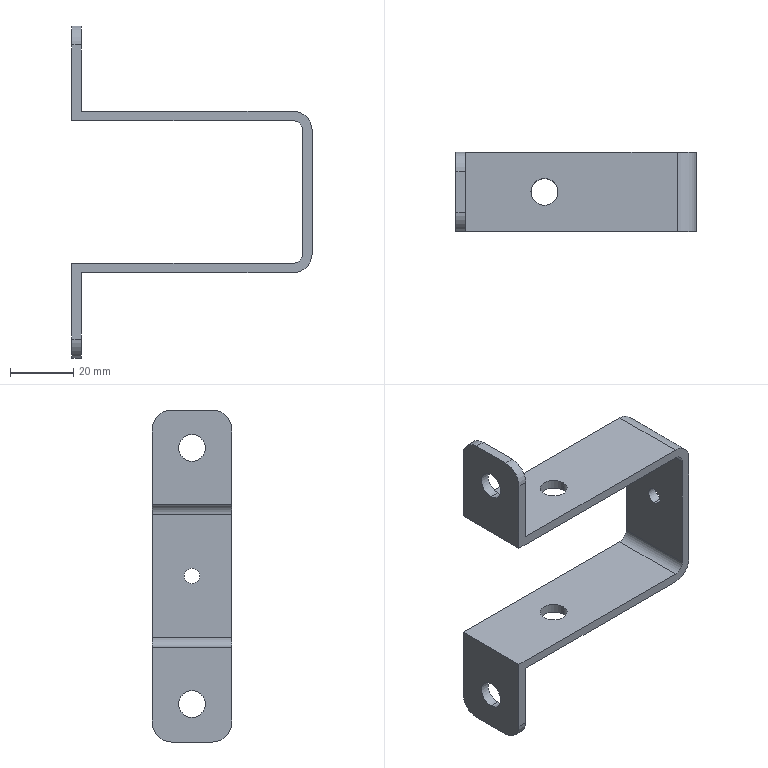Component | SolidWorks | U-shapedFixingBracket-2 | 1 solid | 32 faces | box 76 x 25 x 105 mm | volume 17703 mm3 | cylinder 18 | plane 14 | commonest cylinder face diameters 8.5 x8 12 x6 5 x2 6 x2
build123d program:
from build123d import *

# Parameters (mm, degrees)
BOSS_EXTRUDE1_DEPTH = 25
FILLET2_R           = 6
FILLET3_R           = 3
SKETCH2_R           = 2.5
CUT_EXTRUDE1_DEPTH  = 11
SKETCH3_R           = 4.25
CUT_EXTRUDE2_DEPTH  = 88
SKETCH4_W           = 30
SKETCH4_H           = 25
BOSS_EXTRUDE2_DEPTH = 3
FILLET4_R           = 6
SKETCH5_R           = 4.25
CUT_EXTRUDE3_DEPTH  = 3


with BuildPart() as part:
    # Sketch1 → Boss-Extrude1 (new body)
    with BuildSketch(Plane(origin=(0, 0, 0), x_dir=(1, 0, 0), z_dir=(0, 1, 0))):
        Polygon((0, 0), (0, 73), (51, 73), (51, 0), (48, 0), (48, 70), (3, 70), (3, 0), align=None)
    extrude(amount=BOSS_EXTRUDE1_DEPTH)

    # Fillet2
    fillet2_edges = [part.edges().sort_by_distance(p)[0] for p in [
        (0, 12.5, -73),
        (51, 12.5, -73),
    ]]
    fillet(fillet2_edges, radius=FILLET2_R)

    # Fillet3
    fillet3_edges = [part.edges().sort_by_distance(p)[0] for p in [
        (48, 12.5, -70),
        (3, 12.5, -70),
    ]]
    fillet(fillet3_edges, radius=FILLET3_R)

    # Sketch2 → Cut-Extrude1 (cut)
    with BuildSketch(Plane.XY.offset(-70)):
        with Locations((25.5, 12.5)):
            Circle(SKETCH2_R)
    extrude(amount=-CUT_EXTRUDE1_DEPTH, mode=Mode.SUBTRACT)

    # Sketch3 → Cut-Extrude2 (cut)
    with BuildSketch(Plane.ZY):
        with Locations((-25, 12.5)):
            Circle(SKETCH3_R)
    extrude(amount=-CUT_EXTRUDE2_DEPTH, mode=Mode.SUBTRACT)

    # Sketch4 → Boss-Extrude2 (add)
    with BuildSketch(Plane.XY):
        with Locations((-12, 12.5)):
            Rectangle(SKETCH4_W, SKETCH4_H)
        with Locations((63, 12.5)):
            Rectangle(SKETCH4_W, SKETCH4_H)
    extrude(amount=BOSS_EXTRUDE2_DEPTH)

    # Fillet4
    fillet4_edges = [part.edges().sort_by_distance(p)[0] for p in [
        (-27, 25, 1.5),
        (-27, 0, 1.5),
        (78, 0, 1.5),
        (78, 25, 1.5),
    ]]
    fillet(fillet4_edges, radius=FILLET4_R)

    # Sketch5 → Cut-Extrude3 (cut)
    with BuildSketch(Plane(origin=(0, 0, 0), x_dir=(-1, 0, 0), z_dir=(0, 0, -1))):
        with Locations((15, 12.5)):
            Circle(SKETCH5_R)
        with Locations(Location((-66, 12.5, 0), (0, 0, 180))):
            Circle(SKETCH5_R)
    extrude(amount=-CUT_EXTRUDE3_DEPTH, mode=Mode.SUBTRACT)


solid = part.part

# Placed as in the assembly
solid = solid.moved(Location((-118.793, 489.697, 1830.064), (0, -90, 0)))
STEP:
#1=CARTESIAN_POINT('',(-4.795,19.772,74.481));
#2=VERTEX_POINT('',#1);
#3=CARTESIAN_POINT('',(-4.795,19.772,74.815));
#4=VERTEX_POINT('',#3);
#5=CARTESIAN_POINT('',(-4.795,19.772,74.648));
#6=DIRECTION('',(1.,-0.,0.));
#7=DIRECTION('',(0.,0.,1.));
#8=AXIS2_PLACEMENT_3D('',#5,#6,#7);
#9=CIRCLE('',#8,0.1673);
#10=EDGE_CURVE('',#2,#4,#9,.T.);
#11=ORIENTED_EDGE('',*,*,#10,.F.);
#12=CARTESIAN_POINT('',(-4.677,19.772,74.481));
#13=VERTEX_POINT('',#12);
#14=CARTESIAN_POINT('',(-4.795,19.772,74.481));
#15=DIRECTION('',(1.,-0.,0.));
#16=VECTOR('',#15,39.37);
#17=LINE('',#14,#16);
#18=EDGE_CURVE('',#2,#13,#17,.T.);
#19=ORIENTED_EDGE('',*,*,#18,.T.);
#20=CARTESIAN_POINT('',(-4.677,19.772,74.815));
#21=VERTEX_POINT('',#20);
#22=CARTESIAN_POINT('',(-4.677,19.772,74.648));
#23=DIRECTION('',(1.,-0.,0.));
#24=DIRECTION('',(0.,0.,1.));
#25=AXIS2_PLACEMENT_3D('',#22,#23,#24);
#26=CIRCLE('',#25,0.1673);
#27=EDGE_CURVE('',#13,#21,#26,.T.);
#28=ORIENTED_EDGE('',*,*,#27,.T.);
#29=CARTESIAN_POINT('',(-4.795,19.772,74.815));
#30=DIRECTION('',(1.,-0.,0.));
#31=VECTOR('',#30,39.37);
#32=LINE('',#29,#31);
#33=EDGE_CURVE('',#4,#21,#32,.T.);
#34=ORIENTED_EDGE('',*,*,#33,.F.);
#35=EDGE_LOOP('',(#11,#19,#28,#34));
#36=FACE_OUTER_BOUND('',#35,.T.);
#37=CARTESIAN_POINT('',(-4.795,19.772,74.648));
#38=DIRECTION('',(1.,-0.,0.));
#39=DIRECTION('',(0.,0.,1.));
#40=AXIS2_PLACEMENT_3D('',#37,#38,#39);
#41=CYLINDRICAL_SURFACE('',#40,0.1673);
#42=ADVANCED_FACE('',(#36),#41,.F.);
#43=CARTESIAN_POINT('',(-4.795,19.772,71.292));
#44=VERTEX_POINT('',#43);
#45=CARTESIAN_POINT('',(-4.795,19.772,71.627));
#46=VERTEX_POINT('',#45);
#47=CARTESIAN_POINT('',(-4.795,19.772,71.459));
#48=DIRECTION('',(1.,-0.,0.));
#49=DIRECTION('',(0.,0.,-1.));
#50=AXIS2_PLACEMENT_3D('',#47,#48,#49);
#51=CIRCLE('',#50,0.1673);
#52=EDGE_CURVE('',#44,#46,#51,.T.);
#53=ORIENTED_EDGE('',*,*,#52,.F.);
#54=CARTESIAN_POINT('',(-4.677,19.772,71.292));
#55=VERTEX_POINT('',#54);
#56=CARTESIAN_POINT('',(-4.795,19.772,71.292));
#57=DIRECTION('',(1.,-0.,0.));
#58=VECTOR('',#57,39.37);
#59=LINE('',#56,#58);
#60=EDGE_CURVE('',#44,#55,#59,.T.);
#61=ORIENTED_EDGE('',*,*,#60,.T.);
#62=CARTESIAN_POINT('',(-4.677,19.772,71.627));
#63=VERTEX_POINT('',#62);
#64=CARTESIAN_POINT('',(-4.677,19.772,71.459));
#65=DIRECTION('',(1.,-0.,0.));
#66=DIRECTION('',(0.,0.,-1.));
#67=AXIS2_PLACEMENT_3D('',#64,#65,#66);
#68=CIRCLE('',#67,0.1673);
#69=EDGE_CURVE('',#55,#63,#68,.T.);
#70=ORIENTED_EDGE('',*,*,#69,.T.);
#71=CARTESIAN_POINT('',(-4.795,19.772,71.627));
#72=DIRECTION('',(1.,-0.,0.));
#73=VECTOR('',#72,39.37);
#74=LINE('',#71,#73);
#75=EDGE_CURVE('',#46,#63,#74,.T.);
#76=ORIENTED_EDGE('',*,*,#75,.F.);
#77=EDGE_LOOP('',(#53,#61,#70,#76));
#78=FACE_OUTER_BOUND('',#77,.T.);
#79=CARTESIAN_POINT('',(-4.795,19.772,71.459));
#80=DIRECTION('',(1.,-0.,0.));
#81=DIRECTION('',(0.,0.,1.));
#82=AXIS2_PLACEMENT_3D('',#79,#80,#81);
#83=CYLINDRICAL_SURFACE('',#82,0.1673);
#84=ADVANCED_FACE('',(#78),#83,.F.);
#85=CARTESIAN_POINT('',(-3.525,19.772,72.05));
#86=VERTEX_POINT('',#85);
#87=CARTESIAN_POINT('',(-3.86,19.772,72.05));
#88=VERTEX_POINT('',#87);
#89=CARTESIAN_POINT('',(-3.693,19.772,72.05));
#90=DIRECTION('',(-0.,-0.,1.));
#91=DIRECTION('',(-1.,0.,0.));
#92=AXIS2_PLACEMENT_3D('',#89,#90,#91);
#93=CIRCLE('',#92,0.1673);
#94=EDGE_CURVE('',#86,#88,#93,.T.);
#95=ORIENTED_EDGE('',*,*,#94,.F.);
#96=CARTESIAN_POINT('',(-3.525,19.772,72.168));
#97=VERTEX_POINT('',#96);
#98=CARTESIAN_POINT('',(-3.525,19.772,70.593));
#99=DIRECTION('',(-0.,-0.,1.));
#100=VECTOR('',#99,39.37);
#101=LINE('',#98,#100);
#102=EDGE_CURVE('',#86,#97,#101,.T.);
#103=ORIENTED_EDGE('',*,*,#102,.T.);
#104=CARTESIAN_POINT('',(-3.86,19.772,72.168));
#105=VERTEX_POINT('',#104);
#106=CARTESIAN_POINT('',(-3.693,19.772,72.168));
#107=DIRECTION('',(0.,0.,-1.));
#108=DIRECTION('',(1.,0.,0.));
#109=AXIS2_PLACEMENT_3D('',#106,#107,#108);
#110=CIRCLE('',#109,0.1673);
#111=EDGE_CURVE('',#105,#97,#110,.T.);
#112=ORIENTED_EDGE('',*,*,#111,.F.);
#113=CARTESIAN_POINT('',(-3.86,19.772,70.593));
#114=DIRECTION('',(-0.,-0.,1.));
#115=VECTOR('',#114,39.37);
#116=LINE('',#113,#115);
#117=EDGE_CURVE('',#88,#105,#116,.T.);
#118=ORIENTED_EDGE('',*,*,#117,.F.);
#119=EDGE_LOOP('',(#95,#103,#112,#118));
#120=FACE_OUTER_BOUND('',#119,.T.);
#121=CARTESIAN_POINT('',(-3.693,19.772,70.593));
#122=DIRECTION('',(-0.,-0.,1.));
#123=DIRECTION('',(-1.,0.,0.));
#124=AXIS2_PLACEMENT_3D('',#121,#122,#123);
#125=CYLINDRICAL_SURFACE('',#124,0.1673);
#126=ADVANCED_FACE('',(#120),#125,.F.);
#127=CARTESIAN_POINT('',(-3.525,19.772,73.94));
#128=VERTEX_POINT('',#127);
#129=CARTESIAN_POINT('',(-3.86,19.772,73.94));
#130=VERTEX_POINT('',#129);
#131=CARTESIAN_POINT('',(-3.693,19.772,73.94));
#132=DIRECTION('',(-0.,-0.,1.));
#133=DIRECTION('',(-1.,0.,0.));
#134=AXIS2_PLACEMENT_3D('',#131,#132,#133);
#135=CIRCLE('',#134,0.1673);
#136=EDGE_CURVE('',#128,#130,#135,.T.);
#137=ORIENTED_EDGE('',*,*,#136,.F.);
#138=CARTESIAN_POINT('',(-3.525,19.772,74.058));
#139=VERTEX_POINT('',#138);
#140=CARTESIAN_POINT('',(-3.525,19.772,70.593));
#141=DIRECTION('',(-0.,-0.,1.));
#142=VECTOR('',#141,39.37);
#143=LINE('',#140,#142);
#144=EDGE_CURVE('',#128,#139,#143,.T.);
#145=ORIENTED_EDGE('',*,*,#144,.T.);
#146=CARTESIAN_POINT('',(-3.86,19.772,74.058));
#147=VERTEX_POINT('',#146);
#148=CARTESIAN_POINT('',(-3.693,19.772,74.058));
#149=DIRECTION('',(-0.,-0.,1.));
#150=DIRECTION('',(-1.,0.,0.));
#151=AXIS2_PLACEMENT_3D('',#148,#149,#150);
#152=CIRCLE('',#151,0.1673);
#153=EDGE_CURVE('',#139,#147,#152,.T.);
#154=ORIENTED_EDGE('',*,*,#153,.T.);
#155=CARTESIAN_POINT('',(-3.86,19.772,70.593));
#156=DIRECTION('',(-0.,-0.,1.));
#157=VECTOR('',#156,39.37);
#158=LINE('',#155,#157);
#159=EDGE_CURVE('',#130,#147,#158,.T.);
#160=ORIENTED_EDGE('',*,*,#159,.F.);
#161=EDGE_LOOP('',(#137,#145,#154,#160));
#162=FACE_OUTER_BOUND('',#161,.T.);
#163=CARTESIAN_POINT('',(-3.693,19.772,70.593));
#164=DIRECTION('',(-0.,-0.,1.));
#165=DIRECTION('',(-1.,0.,0.));
#166=AXIS2_PLACEMENT_3D('',#163,#164,#165);
#167=CYLINDRICAL_SURFACE('',#166,0.1673);
#168=ADVANCED_FACE('',(#162),#167,.F.);
#169=CARTESIAN_POINT('',(-1.803,19.772,73.152));
#170=VERTEX_POINT('',#169);
#171=CARTESIAN_POINT('',(-1.803,19.772,72.955));
#172=VERTEX_POINT('',#171);
#173=CARTESIAN_POINT('',(-1.803,19.772,73.054));
#174=DIRECTION('',(-1.,0.,-0.));
#175=DIRECTION('',(0.,0.,-1.));
#176=AXIS2_PLACEMENT_3D('',#173,#174,#175);
#177=CIRCLE('',#176,0.09843);
#178=EDGE_CURVE('',#170,#172,#177,.T.);
#179=ORIENTED_EDGE('',*,*,#178,.F.);
#180=CARTESIAN_POINT('',(-1.921,19.772,73.152));
#181=VERTEX_POINT('',#180);
#182=CARTESIAN_POINT('',(-1.488,19.772,73.152));
#183=DIRECTION('',(-1.,0.,-0.));
#184=VECTOR('',#183,39.37);
#185=LINE('',#182,#184);
#186=EDGE_CURVE('',#170,#181,#185,.T.);
#187=ORIENTED_EDGE('',*,*,#186,.T.);
#188=CARTESIAN_POINT('',(-1.921,19.772,72.955));
#189=VERTEX_POINT('',#188);
#190=CARTESIAN_POINT('',(-1.921,19.772,73.054));
#191=DIRECTION('',(-1.,0.,-0.));
#192=DIRECTION('',(0.,0.,-1.));
#193=AXIS2_PLACEMENT_3D('',#190,#191,#192);
#194=CIRCLE('',#193,0.09843);
#195=EDGE_CURVE('',#181,#189,#194,.T.);
#196=ORIENTED_EDGE('',*,*,#195,.T.);
#197=CARTESIAN_POINT('',(-1.488,19.772,72.955));
#198=DIRECTION('',(-1.,0.,-0.));
#199=VECTOR('',#198,39.37);
#200=LINE('',#197,#199);
#201=EDGE_CURVE('',#172,#189,#200,.T.);
#202=ORIENTED_EDGE('',*,*,#201,.F.);
#203=EDGE_LOOP('',(#179,#187,#196,#202));
#204=FACE_OUTER_BOUND('',#203,.T.);
#205=CARTESIAN_POINT('',(-1.488,19.772,73.054));
#206=DIRECTION('',(-1.,0.,-0.));
#207=DIRECTION('',(0.,0.,-1.));
#208=AXIS2_PLACEMENT_3D('',#205,#206,#207);
#209=CYLINDRICAL_SURFACE('',#208,0.09843);
#210=ADVANCED_FACE('',(#204),#209,.F.);
#211=CARTESIAN_POINT('',(-3.693,19.772,73.94));
#212=DIRECTION('',(-0.,-0.,1.));
#213=DIRECTION('',(-1.,0.,0.));
#214=AXIS2_PLACEMENT_3D('',#211,#212,#213);
#215=CIRCLE('',#214,0.1673);
#216=EDGE_CURVE('',#130,#128,#215,.T.);
#217=ORIENTED_EDGE('',*,*,#216,.T.);
#218=ORIENTED_EDGE('',*,*,#136,.T.);
#219=EDGE_LOOP('',(#217,#218));
#220=FACE_BOUND('',#219,.T.);
#221=CARTESIAN_POINT('',(-4.795,20.264,73.94));
#222=VERTEX_POINT('',#221);
#223=CARTESIAN_POINT('',(-2.039,20.264,73.94));
#224=VERTEX_POINT('',#223);
#225=CARTESIAN_POINT('',(-1.921,20.264,73.94));
#226=DIRECTION('',(1.,-0.,0.));
#227=VECTOR('',#226,39.37);
#228=LINE('',#225,#227);
#229=EDGE_CURVE('',#222,#224,#228,.T.);
#230=ORIENTED_EDGE('',*,*,#229,.T.);
#231=CARTESIAN_POINT('',(-2.039,19.279,73.94));
#232=VERTEX_POINT('',#231);
#233=CARTESIAN_POINT('',(-2.039,19.279,73.94));
#234=DIRECTION('',(-0.,-1.,-0.));
#235=VECTOR('',#234,39.37);
#236=LINE('',#233,#235);
#237=EDGE_CURVE('',#224,#232,#236,.T.);
#238=ORIENTED_EDGE('',*,*,#237,.T.);
#239=CARTESIAN_POINT('',(-4.795,19.279,73.94));
#240=VERTEX_POINT('',#239);
#241=CARTESIAN_POINT('',(-1.921,19.279,73.94));
#242=DIRECTION('',(1.,-0.,0.));
#243=VECTOR('',#242,39.37);
#244=LINE('',#241,#243);
#245=EDGE_CURVE('',#240,#232,#244,.T.);
#246=ORIENTED_EDGE('',*,*,#245,.F.);
#247=CARTESIAN_POINT('',(-4.795,20.264,73.94));
#248=DIRECTION('',(-0.,-1.,-0.));
#249=VECTOR('',#248,39.37);
#250=LINE('',#247,#249);
#251=EDGE_CURVE('',#222,#240,#250,.T.);
#252=ORIENTED_EDGE('',*,*,#251,.F.);
#253=EDGE_LOOP('',(#230,#238,#246,#252));
#254=FACE_OUTER_BOUND('',#253,.T.);
#255=CARTESIAN_POINT('',(-1.921,19.279,73.94));
#256=DIRECTION('',(-0.,-0.,1.));
#257=DIRECTION('',(-1.,0.,-0.));
#258=AXIS2_PLACEMENT_3D('',#255,#256,#257);
#259=PLANE('',#258);
#260=ADVANCED_FACE('',(#220,#254),#259,.F.);
#261=CARTESIAN_POINT('',(-1.921,19.772,73.054));
#262=DIRECTION('',(-1.,0.,-0.));
#263=DIRECTION('',(0.,0.,-1.));
#264=AXIS2_PLACEMENT_3D('',#261,#262,#263);
#265=CIRCLE('',#264,0.09843);
#266=EDGE_CURVE('',#189,#181,#265,.T.);
#267=ORIENTED_EDGE('',*,*,#266,.F.);
#268=ORIENTED_EDGE('',*,*,#195,.F.);
#269=EDGE_LOOP('',(#267,#268));
#270=FACE_BOUND('',#269,.T.);
#271=CARTESIAN_POINT('',(-1.921,20.264,73.821));
#272=VERTEX_POINT('',#271);
#273=CARTESIAN_POINT('',(-1.921,20.264,72.286));
#274=VERTEX_POINT('',#273);
#275=CARTESIAN_POINT('',(-1.921,20.264,72.168));
#276=DIRECTION('',(0.,0.,-1.));
#277=VECTOR('',#276,39.37);
#278=LINE('',#275,#277);
#279=EDGE_CURVE('',#272,#274,#278,.T.);
#280=ORIENTED_EDGE('',*,*,#279,.T.);
#281=CARTESIAN_POINT('',(-1.921,19.279,72.286));
#282=VERTEX_POINT('',#281);
#283=CARTESIAN_POINT('',(-1.921,19.279,72.286));
#284=DIRECTION('',(-0.,-1.,-0.));
#285=VECTOR('',#284,39.37);
#286=LINE('',#283,#285);
#287=EDGE_CURVE('',#274,#282,#286,.T.);
#288=ORIENTED_EDGE('',*,*,#287,.T.);
#289=CARTESIAN_POINT('',(-1.921,19.279,73.821));
#290=VERTEX_POINT('',#289);
#291=CARTESIAN_POINT('',(-1.921,19.279,72.168));
#292=DIRECTION('',(0.,0.,-1.));
#293=VECTOR('',#292,39.37);
#294=LINE('',#291,#293);
#295=EDGE_CURVE('',#290,#282,#294,.T.);
#296=ORIENTED_EDGE('',*,*,#295,.F.);
#297=CARTESIAN_POINT('',(-1.921,20.264,73.821));
#298=DIRECTION('',(0.,1.,0.));
#299=VECTOR('',#298,39.37);
#300=LINE('',#297,#299);
#301=EDGE_CURVE('',#290,#272,#300,.T.);
#302=ORIENTED_EDGE('',*,*,#301,.T.);
#303=EDGE_LOOP('',(#280,#288,#296,#302));
#304=FACE_OUTER_BOUND('',#303,.T.);
#305=CARTESIAN_POINT('',(-1.921,19.279,72.168));
#306=DIRECTION('',(1.,-0.,0.));
#307=DIRECTION('',(-0.,-0.,1.));
#308=AXIS2_PLACEMENT_3D('',#305,#306,#307);
#309=PLANE('',#308);
#310=ADVANCED_FACE('',(#270,#304),#309,.F.);
#311=ORIENTED_EDGE('',*,*,#111,.T.);
#312=CARTESIAN_POINT('',(-3.693,19.772,72.168));
#313=DIRECTION('',(0.,0.,-1.));
#314=DIRECTION('',(1.,0.,0.));
#315=AXIS2_PLACEMENT_3D('',#312,#313,#314);
#316=CIRCLE('',#315,0.1673);
#317=EDGE_CURVE('',#97,#105,#316,.T.);
#318=ORIENTED_EDGE('',*,*,#317,.T.);
#319=EDGE_LOOP('',(#311,#318));
#320=FACE_BOUND('',#319,.T.);
#321=CARTESIAN_POINT('',(-2.039,19.279,72.168));
#322=VERTEX_POINT('',#321);
#323=CARTESIAN_POINT('',(-4.795,19.279,72.168));
#324=VERTEX_POINT('',#323);
#325=CARTESIAN_POINT('',(-4.677,19.279,72.168));
#326=DIRECTION('',(-1.,0.,-0.));
#327=VECTOR('',#326,39.37);
#328=LINE('',#325,#327);
#329=EDGE_CURVE('',#322,#324,#328,.T.);
#330=ORIENTED_EDGE('',*,*,#329,.F.);
#331=CARTESIAN_POINT('',(-2.039,20.264,72.168));
#332=VERTEX_POINT('',#331);
#333=CARTESIAN_POINT('',(-2.039,20.264,72.168));
#334=DIRECTION('',(0.,1.,0.));
#335=VECTOR('',#334,39.37);
#336=LINE('',#333,#335);
#337=EDGE_CURVE('',#322,#332,#336,.T.);
#338=ORIENTED_EDGE('',*,*,#337,.T.);
#339=CARTESIAN_POINT('',(-4.795,20.264,72.168));
#340=VERTEX_POINT('',#339);
#341=CARTESIAN_POINT('',(-4.677,20.264,72.168));
#342=DIRECTION('',(-1.,0.,-0.));
#343=VECTOR('',#342,39.37);
#344=LINE('',#341,#343);
#345=EDGE_CURVE('',#332,#340,#344,.T.);
#346=ORIENTED_EDGE('',*,*,#345,.T.);
#347=CARTESIAN_POINT('',(-4.795,20.264,72.168));
#348=DIRECTION('',(0.,1.,0.));
#349=VECTOR('',#348,39.37);
#350=LINE('',#347,#349);
#351=EDGE_CURVE('',#324,#340,#350,.T.);
#352=ORIENTED_EDGE('',*,*,#351,.F.);
#353=EDGE_LOOP('',(#330,#338,#346,#352));
#354=FACE_OUTER_BOUND('',#353,.T.);
#355=CARTESIAN_POINT('',(-4.677,19.279,72.168));
#356=DIRECTION('',(0.,0.,-1.));
#357=DIRECTION('',(1.,-0.,0.));
#358=AXIS2_PLACEMENT_3D('',#355,#356,#357);
#359=PLANE('',#358);
#360=ADVANCED_FACE('',(#320,#354),#359,.F.);
#361=CARTESIAN_POINT('',(-3.693,19.772,72.05));
#362=DIRECTION('',(-0.,-0.,1.));
#363=DIRECTION('',(-1.,0.,0.));
#364=AXIS2_PLACEMENT_3D('',#361,#362,#363);
#365=CIRCLE('',#364,0.1673);
#366=EDGE_CURVE('',#88,#86,#365,.T.);
#367=ORIENTED_EDGE('',*,*,#366,.T.);
#368=ORIENTED_EDGE('',*,*,#94,.T.);
#369=EDGE_LOOP('',(#367,#368));
#370=FACE_BOUND('',#369,.T.);
#371=CARTESIAN_POINT('',(-4.677,20.264,72.05));
#372=VERTEX_POINT('',#371);
#373=CARTESIAN_POINT('',(-2.039,20.264,72.05));
#374=VERTEX_POINT('',#373);
#375=CARTESIAN_POINT('',(-1.803,20.264,72.05));
#376=DIRECTION('',(1.,-0.,0.));
#377=VECTOR('',#376,39.37);
#378=LINE('',#375,#377);
#379=EDGE_CURVE('',#372,#374,#378,.T.);
#380=ORIENTED_EDGE('',*,*,#379,.T.);
#381=CARTESIAN_POINT('',(-2.039,19.279,72.05));
#382=VERTEX_POINT('',#381);
#383=CARTESIAN_POINT('',(-2.039,19.279,72.05));
#384=DIRECTION('',(-0.,-1.,-0.));
#385=VECTOR('',#384,39.37);
#386=LINE('',#383,#385);
#387=EDGE_CURVE('',#374,#382,#386,.T.);
#388=ORIENTED_EDGE('',*,*,#387,.T.);
#389=CARTESIAN_POINT('',(-4.677,19.279,72.05));
#390=VERTEX_POINT('',#389);
#391=CARTESIAN_POINT('',(-1.803,19.279,72.05));
#392=DIRECTION('',(1.,-0.,0.));
#393=VECTOR('',#392,39.37);
#394=LINE('',#391,#393);
#395=EDGE_CURVE('',#390,#382,#394,.T.);
#396=ORIENTED_EDGE('',*,*,#395,.F.);
#397=CARTESIAN_POINT('',(-4.677,19.279,72.05));
#398=DIRECTION('',(0.,1.,0.));
#399=VECTOR('',#398,39.37);
#400=LINE('',#397,#399);
#401=EDGE_CURVE('',#390,#372,#400,.T.);
#402=ORIENTED_EDGE('',*,*,#401,.T.);
#403=EDGE_LOOP('',(#380,#388,#396,#402));
#404=FACE_OUTER_BOUND('',#403,.T.);
#405=CARTESIAN_POINT('',(-1.803,19.279,72.05));
#406=DIRECTION('',(-0.,-0.,1.));
#407=DIRECTION('',(-1.,0.,-0.));
#408=AXIS2_PLACEMENT_3D('',#405,#406,#407);
#409=PLANE('',#408);
#410=ADVANCED_FACE('',(#370,#404),#409,.F.);
#411=CARTESIAN_POINT('',(-1.803,19.772,73.054));
#412=DIRECTION('',(-1.,0.,-0.));
#413=DIRECTION('',(0.,0.,-1.));
#414=AXIS2_PLACEMENT_3D('',#411,#412,#413);
#415=CIRCLE('',#414,0.09843);
#416=EDGE_CURVE('',#172,#170,#415,.T.);
#417=ORIENTED_EDGE('',*,*,#416,.T.);
#418=ORIENTED_EDGE('',*,*,#178,.T.);
#419=EDGE_LOOP('',(#417,#418));
#420=FACE_BOUND('',#419,.T.);
#421=CARTESIAN_POINT('',(-1.803,19.279,72.286));
#422=VERTEX_POINT('',#421);
#423=CARTESIAN_POINT('',(-1.803,19.279,73.821));
#424=VERTEX_POINT('',#423);
#425=CARTESIAN_POINT('',(-1.803,19.279,74.058));
#426=DIRECTION('',(-0.,-0.,1.));
#427=VECTOR('',#426,39.37);
#428=LINE('',#425,#427);
#429=EDGE_CURVE('',#422,#424,#428,.T.);
#430=ORIENTED_EDGE('',*,*,#429,.F.);
#431=CARTESIAN_POINT('',(-1.803,20.264,72.286));
#432=VERTEX_POINT('',#431);
#433=CARTESIAN_POINT('',(-1.803,19.279,72.286));
#434=DIRECTION('',(0.,1.,0.));
#435=VECTOR('',#434,39.37);
#436=LINE('',#433,#435);
#437=EDGE_CURVE('',#422,#432,#436,.T.);
#438=ORIENTED_EDGE('',*,*,#437,.T.);
#439=CARTESIAN_POINT('',(-1.803,20.264,73.821));
#440=VERTEX_POINT('',#439);
#441=CARTESIAN_POINT('',(-1.803,20.264,74.058));
#442=DIRECTION('',(-0.,-0.,1.));
#443=VECTOR('',#442,39.37);
#444=LINE('',#441,#443);
#445=EDGE_CURVE('',#432,#440,#444,.T.);
#446=ORIENTED_EDGE('',*,*,#445,.T.);
#447=CARTESIAN_POINT('',(-1.803,19.279,73.821));
#448=DIRECTION('',(-0.,-1.,-0.));
#449=VECTOR('',#448,39.37);
#450=LINE('',#447,#449);
#451=EDGE_CURVE('',#440,#424,#450,.T.);
#452=ORIENTED_EDGE('',*,*,#451,.T.);
#453=EDGE_LOOP('',(#430,#438,#446,#452));
#454=FACE_OUTER_BOUND('',#453,.T.);
#455=CARTESIAN_POINT('',(-1.803,19.279,74.058));
#456=DIRECTION('',(-1.,0.,-0.));
#457=DIRECTION('',(0.,0.,-1.));
#458=AXIS2_PLACEMENT_3D('',#455,#456,#457);
#459=PLANE('',#458);
#460=ADVANCED_FACE('',(#420,#454),#459,.F.);
#461=CARTESIAN_POINT('',(-3.693,19.772,74.058));
#462=DIRECTION('',(-0.,-0.,1.));
#463=DIRECTION('',(-1.,0.,0.));
#464=AXIS2_PLACEMENT_3D('',#461,#462,#463);
#465=CIRCLE('',#464,0.1673);
#466=EDGE_CURVE('',#147,#139,#465,.T.);
#467=ORIENTED_EDGE('',*,*,#466,.F.);
#468=ORIENTED_EDGE('',*,*,#153,.F.);
#469=EDGE_LOOP('',(#467,#468));
#470=FACE_BOUND('',#469,.T.);
#471=CARTESIAN_POINT('',(-2.039,19.279,74.058));
#472=VERTEX_POINT('',#471);
#473=CARTESIAN_POINT('',(-4.677,19.279,74.058));
#474=VERTEX_POINT('',#473);
#475=CARTESIAN_POINT('',(-4.677,19.279,74.058));
#476=DIRECTION('',(-1.,0.,-0.));
#477=VECTOR('',#476,39.37);
#478=LINE('',#475,#477);
#479=EDGE_CURVE('',#472,#474,#478,.T.);
#480=ORIENTED_EDGE('',*,*,#479,.F.);
#481=CARTESIAN_POINT('',(-2.039,20.264,74.058));
#482=VERTEX_POINT('',#481);
#483=CARTESIAN_POINT('',(-2.039,19.279,74.058));
#484=DIRECTION('',(0.,1.,0.));
#485=VECTOR('',#484,39.37);
#486=LINE('',#483,#485);
#487=EDGE_CURVE('',#472,#482,#486,.T.);
#488=ORIENTED_EDGE('',*,*,#487,.T.);
#489=CARTESIAN_POINT('',(-4.677,20.264,74.058));
#490=VERTEX_POINT('',#489);
#491=CARTESIAN_POINT('',(-4.677,20.264,74.058));
#492=DIRECTION('',(-1.,0.,-0.));
#493=VECTOR('',#492,39.37);
#494=LINE('',#491,#493);
#495=EDGE_CURVE('',#482,#490,#494,.T.);
#496=ORIENTED_EDGE('',*,*,#495,.T.);
#497=CARTESIAN_POINT('',(-4.677,19.279,74.058));
#498=DIRECTION('',(0.,1.,0.));
#499=VECTOR('',#498,39.37);
#500=LINE('',#497,#499);
#501=EDGE_CURVE('',#474,#490,#500,.T.);
#502=ORIENTED_EDGE('',*,*,#501,.F.);
#503=EDGE_LOOP('',(#480,#488,#496,#502));
#504=FACE_OUTER_BOUND('',#503,.T.);
#505=CARTESIAN_POINT('',(-4.677,19.279,74.058));
#506=DIRECTION('',(0.,0.,-1.));
#507=DIRECTION('',(1.,-0.,0.));
#508=AXIS2_PLACEMENT_3D('',#505,#506,#507);
#509=PLANE('',#508);
#510=ADVANCED_FACE('',(#470,#504),#509,.F.);
#511=CARTESIAN_POINT('',(-4.795,19.279,71.223));
#512=VERTEX_POINT('',#511);
#513=CARTESIAN_POINT('',(-4.795,19.279,72.168));
#514=DIRECTION('',(-0.,-0.,1.));
#515=VECTOR('',#514,39.37);
#516=LINE('',#513,#515);
#517=EDGE_CURVE('',#512,#324,#516,.T.);
#518=ORIENTED_EDGE('',*,*,#517,.F.);
#519=CARTESIAN_POINT('',(-4.677,19.279,71.223));
#520=VERTEX_POINT('',#519);
#521=CARTESIAN_POINT('',(-4.677,19.279,71.223));
#522=DIRECTION('',(1.,-0.,0.));
#523=VECTOR('',#522,39.37);
#524=LINE('',#521,#523);
#525=EDGE_CURVE('',#512,#520,#524,.T.);
#526=ORIENTED_EDGE('',*,*,#525,.T.);
#527=CARTESIAN_POINT('',(-4.677,19.279,72.168));
#528=DIRECTION('',(-0.,-0.,1.));
#529=VECTOR('',#528,39.37);
#530=LINE('',#527,#529);
#531=EDGE_CURVE('',#520,#390,#530,.T.);
#532=ORIENTED_EDGE('',*,*,#531,.T.);
#533=ORIENTED_EDGE('',*,*,#395,.T.);
#534=CARTESIAN_POINT('',(-2.039,19.279,72.286));
#535=DIRECTION('',(-0.,-1.,-0.));
#536=DIRECTION('',(1.,0.,0.));
#537=AXIS2_PLACEMENT_3D('',#534,#535,#536);
#538=CIRCLE('',#537,0.2362);
#539=EDGE_CURVE('',#382,#422,#538,.T.);
#540=ORIENTED_EDGE('',*,*,#539,.T.);
#541=ORIENTED_EDGE('',*,*,#429,.T.);
#542=CARTESIAN_POINT('',(-2.039,19.279,73.821));
#543=DIRECTION('',(-0.,-1.,-0.));
#544=DIRECTION('',(1.,0.,0.));
#545=AXIS2_PLACEMENT_3D('',#542,#543,#544);
#546=CIRCLE('',#545,0.2362);
#547=EDGE_CURVE('',#424,#472,#546,.T.);
#548=ORIENTED_EDGE('',*,*,#547,.T.);
#549=ORIENTED_EDGE('',*,*,#479,.T.);
#550=CARTESIAN_POINT('',(-4.677,19.279,74.884));
#551=VERTEX_POINT('',#550);
#552=CARTESIAN_POINT('',(-4.677,19.279,73.94));
#553=DIRECTION('',(-0.,0.,1.));
#554=VECTOR('',#553,39.37);
#555=LINE('',#552,#554);
#556=EDGE_CURVE('',#474,#551,#555,.T.);
#557=ORIENTED_EDGE('',*,*,#556,.T.);
#558=CARTESIAN_POINT('',(-4.795,19.279,74.884));
#559=VERTEX_POINT('',#558);
#560=CARTESIAN_POINT('',(-4.677,19.279,74.884));
#561=DIRECTION('',(-1.,0.,-0.));
#562=VECTOR('',#561,39.37);
#563=LINE('',#560,#562);
#564=EDGE_CURVE('',#551,#559,#563,.T.);
#565=ORIENTED_EDGE('',*,*,#564,.T.);
#566=CARTESIAN_POINT('',(-4.795,19.279,73.94));
#567=DIRECTION('',(-0.,0.,1.));
#568=VECTOR('',#567,39.37);
#569=LINE('',#566,#568);
#570=EDGE_CURVE('',#240,#559,#569,.T.);
#571=ORIENTED_EDGE('',*,*,#570,.F.);
#572=ORIENTED_EDGE('',*,*,#245,.T.);
#573=CARTESIAN_POINT('',(-2.039,19.279,73.821));
#574=DIRECTION('',(0.,1.,0.));
#575=DIRECTION('',(1.,0.,0.));
#576=AXIS2_PLACEMENT_3D('',#573,#574,#575);
#577=CIRCLE('',#576,0.1181);
#578=EDGE_CURVE('',#232,#290,#577,.T.);
#579=ORIENTED_EDGE('',*,*,#578,.T.);
#580=ORIENTED_EDGE('',*,*,#295,.T.);
#581=CARTESIAN_POINT('',(-2.039,19.279,72.286));
#582=DIRECTION('',(0.,1.,0.));
#583=DIRECTION('',(1.,0.,0.));
#584=AXIS2_PLACEMENT_3D('',#581,#582,#583);
#585=CIRCLE('',#584,0.1181);
#586=EDGE_CURVE('',#282,#322,#585,.T.);
#587=ORIENTED_EDGE('',*,*,#586,.T.);
#588=ORIENTED_EDGE('',*,*,#329,.T.);
#589=EDGE_LOOP('',(#518,#526,#532,#533,#540,#541,#548,#549,#557,#565,#571,#572,#579,#580,#587,#588));
#590=FACE_OUTER_BOUND('',#589,.T.);
#591=CARTESIAN_POINT('',(-4.677,19.279,74.058));
#592=DIRECTION('',(0.,1.,0.));
#593=DIRECTION('',(1.,-0.,0.));
#594=AXIS2_PLACEMENT_3D('',#591,#592,#593);
#595=PLANE('',#594);
#596=ADVANCED_FACE('',(#590),#595,.F.);
#597=CARTESIAN_POINT('',(-4.677,20.264,71.223));
#598=VERTEX_POINT('',#597);
#599=CARTESIAN_POINT('',(-4.677,20.264,70.987));
#600=DIRECTION('',(0.,0.,-1.));
#601=VECTOR('',#600,39.37);
#602=LINE('',#599,#601);
#603=EDGE_CURVE('',#372,#598,#602,.T.);
#604=ORIENTED_EDGE('',*,*,#603,.T.);
#605=CARTESIAN_POINT('',(-4.795,20.264,71.223));
#606=VERTEX_POINT('',#605);
#607=CARTESIAN_POINT('',(-4.795,20.264,71.223));
#608=DIRECTION('',(-1.,0.,-0.));
#609=VECTOR('',#608,39.37);
#610=LINE('',#607,#609);
#611=EDGE_CURVE('',#598,#606,#610,.T.);
#612=ORIENTED_EDGE('',*,*,#611,.T.);
#613=CARTESIAN_POINT('',(-4.795,20.264,70.987));
#614=DIRECTION('',(0.,0.,-1.));
#615=VECTOR('',#614,39.37);
#616=LINE('',#613,#615);
#617=EDGE_CURVE('',#340,#606,#616,.T.);
#618=ORIENTED_EDGE('',*,*,#617,.F.);
#619=ORIENTED_EDGE('',*,*,#345,.F.);
#620=CARTESIAN_POINT('',(-2.039,20.264,72.286));
#621=DIRECTION('',(-0.,-1.,-0.));
#622=DIRECTION('',(1.,0.,0.));
#623=AXIS2_PLACEMENT_3D('',#620,#621,#622);
#624=CIRCLE('',#623,0.1181);
#625=EDGE_CURVE('',#332,#274,#624,.T.);
#626=ORIENTED_EDGE('',*,*,#625,.T.);
#627=ORIENTED_EDGE('',*,*,#279,.F.);
#628=CARTESIAN_POINT('',(-2.039,20.264,73.821));
#629=DIRECTION('',(-0.,-1.,-0.));
#630=DIRECTION('',(1.,0.,0.));
#631=AXIS2_PLACEMENT_3D('',#628,#629,#630);
#632=CIRCLE('',#631,0.1181);
#633=EDGE_CURVE('',#272,#224,#632,.T.);
#634=ORIENTED_EDGE('',*,*,#633,.T.);
#635=ORIENTED_EDGE('',*,*,#229,.F.);
#636=CARTESIAN_POINT('',(-4.795,20.264,74.884));
#637=VERTEX_POINT('',#636);
#638=CARTESIAN_POINT('',(-4.795,20.264,75.121));
#639=DIRECTION('',(0.,0.,-1.));
#640=VECTOR('',#639,39.37);
#641=LINE('',#638,#640);
#642=EDGE_CURVE('',#637,#222,#641,.T.);
#643=ORIENTED_EDGE('',*,*,#642,.F.);
#644=CARTESIAN_POINT('',(-4.677,20.264,74.884));
#645=VERTEX_POINT('',#644);
#646=CARTESIAN_POINT('',(-4.677,20.264,74.884));
#647=DIRECTION('',(1.,-0.,0.));
#648=VECTOR('',#647,39.37);
#649=LINE('',#646,#648);
#650=EDGE_CURVE('',#637,#645,#649,.T.);
#651=ORIENTED_EDGE('',*,*,#650,.T.);
#652=CARTESIAN_POINT('',(-4.677,20.264,75.121));
#653=DIRECTION('',(0.,0.,-1.));
#654=VECTOR('',#653,39.37);
#655=LINE('',#652,#654);
#656=EDGE_CURVE('',#645,#490,#655,.T.);
#657=ORIENTED_EDGE('',*,*,#656,.T.);
#658=ORIENTED_EDGE('',*,*,#495,.F.);
#659=CARTESIAN_POINT('',(-2.039,20.264,73.821));
#660=DIRECTION('',(0.,1.,0.));
#661=DIRECTION('',(1.,0.,0.));
#662=AXIS2_PLACEMENT_3D('',#659,#660,#661);
#663=CIRCLE('',#662,0.2362);
#664=EDGE_CURVE('',#482,#440,#663,.T.);
#665=ORIENTED_EDGE('',*,*,#664,.T.);
#666=ORIENTED_EDGE('',*,*,#445,.F.);
#667=CARTESIAN_POINT('',(-2.039,20.264,72.286));
#668=DIRECTION('',(0.,1.,0.));
#669=DIRECTION('',(1.,0.,0.));
#670=AXIS2_PLACEMENT_3D('',#667,#668,#669);
#671=CIRCLE('',#670,0.2362);
#672=EDGE_CURVE('',#432,#374,#671,.T.);
#673=ORIENTED_EDGE('',*,*,#672,.T.);
#674=ORIENTED_EDGE('',*,*,#379,.F.);
#675=EDGE_LOOP('',(#604,#612,#618,#619,#626,#627,#634,#635,#643,#651,#657,#658,#665,#666,#673,#674));
#676=FACE_OUTER_BOUND('',#675,.T.);
#677=CARTESIAN_POINT('',(-4.677,20.264,74.058));
#678=DIRECTION('',(0.,1.,0.));
#679=DIRECTION('',(1.,-0.,0.));
#680=AXIS2_PLACEMENT_3D('',#677,#678,#679);
#681=PLANE('',#680);
#682=ADVANCED_FACE('',(#676),#681,.T.);
#683=ORIENTED_EDGE('',*,*,#539,.F.);
#684=ORIENTED_EDGE('',*,*,#387,.F.);
#685=ORIENTED_EDGE('',*,*,#672,.F.);
#686=ORIENTED_EDGE('',*,*,#437,.F.);
#687=EDGE_LOOP('',(#683,#684,#685,#686));
#688=FACE_OUTER_BOUND('',#687,.T.);
#689=CARTESIAN_POINT('',(-2.039,19.279,72.286));
#690=DIRECTION('',(0.,1.,0.));
#691=DIRECTION('',(1.,0.,0.));
#692=AXIS2_PLACEMENT_3D('',#689,#690,#691);
#693=CYLINDRICAL_SURFACE('',#692,0.2362);
#694=ADVANCED_FACE('',(#688),#693,.T.);
#695=ORIENTED_EDGE('',*,*,#547,.F.);
#696=ORIENTED_EDGE('',*,*,#451,.F.);
#697=ORIENTED_EDGE('',*,*,#664,.F.);
#698=ORIENTED_EDGE('',*,*,#487,.F.);
#699=EDGE_LOOP('',(#695,#696,#697,#698));
#700=FACE_OUTER_BOUND('',#699,.T.);
#701=CARTESIAN_POINT('',(-2.039,19.279,73.821));
#702=DIRECTION('',(0.,1.,0.));
#703=DIRECTION('',(1.,0.,0.));
#704=AXIS2_PLACEMENT_3D('',#701,#702,#703);
#705=CYLINDRICAL_SURFACE('',#704,0.2362);
#706=ADVANCED_FACE('',(#700),#705,.T.);
#707=ORIENTED_EDGE('',*,*,#586,.F.);
#708=ORIENTED_EDGE('',*,*,#287,.F.);
#709=ORIENTED_EDGE('',*,*,#625,.F.);
#710=ORIENTED_EDGE('',*,*,#337,.F.);
#711=EDGE_LOOP('',(#707,#708,#709,#710));
#712=FACE_OUTER_BOUND('',#711,.T.);
#713=CARTESIAN_POINT('',(-2.039,19.279,72.286));
#714=DIRECTION('',(-0.,-1.,-0.));
#715=DIRECTION('',(-1.,0.,0.));
#716=AXIS2_PLACEMENT_3D('',#713,#714,#715);
#717=CYLINDRICAL_SURFACE('',#716,0.1181);
#718=ADVANCED_FACE('',(#712),#717,.F.);
#719=ORIENTED_EDGE('',*,*,#578,.F.);
#720=ORIENTED_EDGE('',*,*,#237,.F.);
#721=ORIENTED_EDGE('',*,*,#633,.F.);
#722=ORIENTED_EDGE('',*,*,#301,.F.);
#723=EDGE_LOOP('',(#719,#720,#721,#722));
#724=FACE_OUTER_BOUND('',#723,.T.);
#725=CARTESIAN_POINT('',(-2.039,19.279,73.821));
#726=DIRECTION('',(-0.,-1.,-0.));
#727=DIRECTION('',(-1.,0.,0.));
#728=AXIS2_PLACEMENT_3D('',#725,#726,#727);
#729=CYLINDRICAL_SURFACE('',#728,0.1181);
#730=ADVANCED_FACE('',(#724),#729,.F.);
#731=ORIENTED_EDGE('',*,*,#186,.F.);
#732=ORIENTED_EDGE('',*,*,#416,.F.);
#733=ORIENTED_EDGE('',*,*,#201,.T.);
#734=ORIENTED_EDGE('',*,*,#266,.T.);
#735=EDGE_LOOP('',(#731,#732,#733,#734));
#736=FACE_OUTER_BOUND('',#735,.T.);
#737=CARTESIAN_POINT('',(-1.488,19.772,73.054));
#738=DIRECTION('',(-1.,0.,-0.));
#739=DIRECTION('',(0.,0.,-1.));
#740=AXIS2_PLACEMENT_3D('',#737,#738,#739);
#741=CYLINDRICAL_SURFACE('',#740,0.09843);
#742=ADVANCED_FACE('',(#736),#741,.F.);
#743=ORIENTED_EDGE('',*,*,#144,.F.);
#744=ORIENTED_EDGE('',*,*,#216,.F.);
#745=ORIENTED_EDGE('',*,*,#159,.T.);
#746=ORIENTED_EDGE('',*,*,#466,.T.);
#747=EDGE_LOOP('',(#743,#744,#745,#746));
#748=FACE_OUTER_BOUND('',#747,.T.);
#749=CARTESIAN_POINT('',(-3.693,19.772,70.593));
#750=DIRECTION('',(-0.,-0.,1.));
#751=DIRECTION('',(-1.,0.,0.));
#752=AXIS2_PLACEMENT_3D('',#749,#750,#751);
#753=CYLINDRICAL_SURFACE('',#752,0.1673);
#754=ADVANCED_FACE('',(#748),#753,.F.);
#755=ORIENTED_EDGE('',*,*,#102,.F.);
#756=ORIENTED_EDGE('',*,*,#366,.F.);
#757=ORIENTED_EDGE('',*,*,#117,.T.);
#758=ORIENTED_EDGE('',*,*,#317,.F.);
#759=EDGE_LOOP('',(#755,#756,#757,#758));
#760=FACE_OUTER_BOUND('',#759,.T.);
#761=CARTESIAN_POINT('',(-3.693,19.772,70.593));
#762=DIRECTION('',(-0.,-0.,1.));
#763=DIRECTION('',(-1.,0.,0.));
#764=AXIS2_PLACEMENT_3D('',#761,#762,#763);
#765=CYLINDRICAL_SURFACE('',#764,0.1673);
#766=ADVANCED_FACE('',(#760),#765,.F.);
#767=CARTESIAN_POINT('',(-4.677,19.772,74.648));
#768=DIRECTION('',(1.,-0.,0.));
#769=DIRECTION('',(0.,0.,1.));
#770=AXIS2_PLACEMENT_3D('',#767,#768,#769);
#771=CIRCLE('',#770,0.1673);
#772=EDGE_CURVE('',#21,#13,#771,.T.);
#773=ORIENTED_EDGE('',*,*,#772,.F.);
#774=ORIENTED_EDGE('',*,*,#27,.F.);
#775=EDGE_LOOP('',(#773,#774));
#776=FACE_BOUND('',#775,.T.);
#777=ORIENTED_EDGE('',*,*,#656,.F.);
#778=CARTESIAN_POINT('',(-4.677,20.027,75.121));
#779=VERTEX_POINT('',#778);
#780=CARTESIAN_POINT('',(-4.677,20.027,74.884));
#781=DIRECTION('',(1.,-0.,0.));
#782=DIRECTION('',(0.,0.,-1.));
#783=AXIS2_PLACEMENT_3D('',#780,#781,#782);
#784=CIRCLE('',#783,0.2362);
#785=EDGE_CURVE('',#645,#779,#784,.T.);
#786=ORIENTED_EDGE('',*,*,#785,.T.);
#787=CARTESIAN_POINT('',(-4.677,19.516,75.121));
#788=VERTEX_POINT('',#787);
#789=CARTESIAN_POINT('',(-4.677,19.279,75.121));
#790=DIRECTION('',(0.,1.,-0.));
#791=VECTOR('',#790,39.37);
#792=LINE('',#789,#791);
#793=EDGE_CURVE('',#788,#779,#792,.T.);
#794=ORIENTED_EDGE('',*,*,#793,.F.);
#795=CARTESIAN_POINT('',(-4.677,19.516,74.884));
#796=DIRECTION('',(1.,-0.,0.));
#797=DIRECTION('',(0.,0.,-1.));
#798=AXIS2_PLACEMENT_3D('',#795,#796,#797);
#799=CIRCLE('',#798,0.2362);
#800=EDGE_CURVE('',#788,#551,#799,.T.);
#801=ORIENTED_EDGE('',*,*,#800,.T.);
#802=ORIENTED_EDGE('',*,*,#556,.F.);
#803=ORIENTED_EDGE('',*,*,#501,.T.);
#804=EDGE_LOOP('',(#777,#786,#794,#801,#802,#803));
#805=FACE_OUTER_BOUND('',#804,.T.);
#806=CARTESIAN_POINT('',(-4.677,20.264,74.058));
#807=DIRECTION('',(-1.,0.,-0.));
#808=DIRECTION('',(0.,0.,-1.));
#809=AXIS2_PLACEMENT_3D('',#806,#807,#808);
#810=PLANE('',#809);
#811=ADVANCED_FACE('',(#776,#805),#810,.F.);
#812=ORIENTED_EDGE('',*,*,#793,.T.);
#813=CARTESIAN_POINT('',(-4.795,20.027,75.121));
#814=VERTEX_POINT('',#813);
#815=CARTESIAN_POINT('',(-4.795,20.027,75.121));
#816=DIRECTION('',(-1.,0.,-0.));
#817=VECTOR('',#816,39.37);
#818=LINE('',#815,#817);
#819=EDGE_CURVE('',#779,#814,#818,.T.);
#820=ORIENTED_EDGE('',*,*,#819,.T.);
#821=CARTESIAN_POINT('',(-4.795,19.516,75.121));
#822=VERTEX_POINT('',#821);
#823=CARTESIAN_POINT('',(-4.795,19.279,75.121));
#824=DIRECTION('',(0.,1.,-0.));
#825=VECTOR('',#824,39.37);
#826=LINE('',#823,#825);
#827=EDGE_CURVE('',#822,#814,#826,.T.);
#828=ORIENTED_EDGE('',*,*,#827,.F.);
#829=CARTESIAN_POINT('',(-4.795,19.516,75.121));
#830=DIRECTION('',(1.,-0.,0.));
#831=VECTOR('',#830,39.37);
#832=LINE('',#829,#831);
#833=EDGE_CURVE('',#822,#788,#832,.T.);
#834=ORIENTED_EDGE('',*,*,#833,.T.);
#835=EDGE_LOOP('',(#812,#820,#828,#834));
#836=FACE_OUTER_BOUND('',#835,.T.);
#837=CARTESIAN_POINT('',(-4.795,19.279,75.121));
#838=DIRECTION('',(0.,-0.,-1.));
#839=DIRECTION('',(-0.,-1.,0.));
#840=AXIS2_PLACEMENT_3D('',#837,#838,#839);
#841=PLANE('',#840);
#842=ADVANCED_FACE('',(#836),#841,.F.);
#843=CARTESIAN_POINT('',(-4.795,19.772,74.648));
#844=DIRECTION('',(1.,-0.,0.));
#845=DIRECTION('',(0.,0.,1.));
#846=AXIS2_PLACEMENT_3D('',#843,#844,#845);
#847=CIRCLE('',#846,0.1673);
#848=EDGE_CURVE('',#4,#2,#847,.T.);
#849=ORIENTED_EDGE('',*,*,#848,.T.);
#850=ORIENTED_EDGE('',*,*,#10,.T.);
#851=EDGE_LOOP('',(#849,#850));
#852=FACE_BOUND('',#851,.T.);
#853=ORIENTED_EDGE('',*,*,#827,.T.);
#854=CARTESIAN_POINT('',(-4.795,20.027,74.884));
#855=DIRECTION('',(-1.,0.,-0.));
#856=DIRECTION('',(0.,0.,-1.));
#857=AXIS2_PLACEMENT_3D('',#854,#855,#856);
#858=CIRCLE('',#857,0.2362);
#859=EDGE_CURVE('',#814,#637,#858,.T.);
#860=ORIENTED_EDGE('',*,*,#859,.T.);
#861=ORIENTED_EDGE('',*,*,#642,.T.);
#862=ORIENTED_EDGE('',*,*,#251,.T.);
#863=ORIENTED_EDGE('',*,*,#570,.T.);
#864=CARTESIAN_POINT('',(-4.795,19.516,74.884));
#865=DIRECTION('',(-1.,0.,-0.));
#866=DIRECTION('',(0.,0.,-1.));
#867=AXIS2_PLACEMENT_3D('',#864,#865,#866);
#868=CIRCLE('',#867,0.2362);
#869=EDGE_CURVE('',#559,#822,#868,.T.);
#870=ORIENTED_EDGE('',*,*,#869,.T.);
#871=EDGE_LOOP('',(#853,#860,#861,#862,#863,#870));
#872=FACE_OUTER_BOUND('',#871,.T.);
#873=CARTESIAN_POINT('',(-4.795,20.264,74.058));
#874=DIRECTION('',(-1.,0.,-0.));
#875=DIRECTION('',(0.,0.,-1.));
#876=AXIS2_PLACEMENT_3D('',#873,#874,#875);
#877=PLANE('',#876);
#878=ADVANCED_FACE('',(#852,#872),#877,.T.);
#879=CARTESIAN_POINT('',(-4.677,19.772,71.459));
#880=DIRECTION('',(1.,-0.,0.));
#881=DIRECTION('',(0.,0.,-1.));
#882=AXIS2_PLACEMENT_3D('',#879,#880,#881);
#883=CIRCLE('',#882,0.1673);
#884=EDGE_CURVE('',#63,#55,#883,.T.);
#885=ORIENTED_EDGE('',*,*,#884,.F.);
#886=ORIENTED_EDGE('',*,*,#69,.F.);
#887=EDGE_LOOP('',(#885,#886));
#888=FACE_BOUND('',#887,.T.);
#889=CARTESIAN_POINT('',(-4.677,20.027,70.987));
#890=VERTEX_POINT('',#889);
#891=CARTESIAN_POINT('',(-4.677,19.516,70.987));
#892=VERTEX_POINT('',#891);
#893=CARTESIAN_POINT('',(-4.677,19.279,70.987));
#894=DIRECTION('',(-0.,-1.,-0.));
#895=VECTOR('',#894,39.37);
#896=LINE('',#893,#895);
#897=EDGE_CURVE('',#890,#892,#896,.T.);
#898=ORIENTED_EDGE('',*,*,#897,.F.);
#899=CARTESIAN_POINT('',(-4.677,20.027,71.223));
#900=DIRECTION('',(1.,-0.,0.));
#901=DIRECTION('',(0.,0.,1.));
#902=AXIS2_PLACEMENT_3D('',#899,#900,#901);
#903=CIRCLE('',#902,0.2362);
#904=EDGE_CURVE('',#890,#598,#903,.T.);
#905=ORIENTED_EDGE('',*,*,#904,.T.);
#906=ORIENTED_EDGE('',*,*,#603,.F.);
#907=ORIENTED_EDGE('',*,*,#401,.F.);
#908=ORIENTED_EDGE('',*,*,#531,.F.);
#909=CARTESIAN_POINT('',(-4.677,19.516,71.223));
#910=DIRECTION('',(1.,-0.,0.));
#911=DIRECTION('',(0.,0.,1.));
#912=AXIS2_PLACEMENT_3D('',#909,#910,#911);
#913=CIRCLE('',#912,0.2362);
#914=EDGE_CURVE('',#520,#892,#913,.T.);
#915=ORIENTED_EDGE('',*,*,#914,.T.);
#916=EDGE_LOOP('',(#898,#905,#906,#907,#908,#915));
#917=FACE_OUTER_BOUND('',#916,.T.);
#918=CARTESIAN_POINT('',(-4.677,20.264,74.058));
#919=DIRECTION('',(1.,-0.,0.));
#920=DIRECTION('',(-0.,-0.,1.));
#921=AXIS2_PLACEMENT_3D('',#918,#919,#920);
#922=PLANE('',#921);
#923=ADVANCED_FACE('',(#888,#917),#922,.T.);
#924=CARTESIAN_POINT('',(-4.795,20.027,70.987));
#925=VERTEX_POINT('',#924);
#926=CARTESIAN_POINT('',(-4.795,19.516,70.987));
#927=VERTEX_POINT('',#926);
#928=CARTESIAN_POINT('',(-4.795,19.279,70.987));
#929=DIRECTION('',(-0.,-1.,-0.));
#930=VECTOR('',#929,39.37);
#931=LINE('',#928,#930);
#932=EDGE_CURVE('',#925,#927,#931,.T.);
#933=ORIENTED_EDGE('',*,*,#932,.F.);
#934=CARTESIAN_POINT('',(-4.677,20.027,70.987));
#935=DIRECTION('',(1.,-0.,0.));
#936=VECTOR('',#935,39.37);
#937=LINE('',#934,#936);
#938=EDGE_CURVE('',#925,#890,#937,.T.);
#939=ORIENTED_EDGE('',*,*,#938,.T.);
#940=ORIENTED_EDGE('',*,*,#897,.T.);
#941=CARTESIAN_POINT('',(-4.795,19.516,70.987));
#942=DIRECTION('',(-1.,0.,-0.));
#943=VECTOR('',#942,39.37);
#944=LINE('',#941,#943);
#945=EDGE_CURVE('',#892,#927,#944,.T.);
#946=ORIENTED_EDGE('',*,*,#945,.T.);
#947=EDGE_LOOP('',(#933,#939,#940,#946));
#948=FACE_OUTER_BOUND('',#947,.T.);
#949=CARTESIAN_POINT('',(-4.795,19.279,70.987));
#950=DIRECTION('',(-0.,-0.,1.));
#951=DIRECTION('',(-1.,0.,-0.));
#952=AXIS2_PLACEMENT_3D('',#949,#950,#951);
#953=PLANE('',#952);
#954=ADVANCED_FACE('',(#948),#953,.F.);
#955=CARTESIAN_POINT('',(-4.795,19.772,71.459));
#956=DIRECTION('',(1.,-0.,0.));
#957=DIRECTION('',(0.,0.,-1.));
#958=AXIS2_PLACEMENT_3D('',#955,#956,#957);
#959=CIRCLE('',#958,0.1673);
#960=EDGE_CURVE('',#46,#44,#959,.T.);
#961=ORIENTED_EDGE('',*,*,#960,.T.);
#962=ORIENTED_EDGE('',*,*,#52,.T.);
#963=EDGE_LOOP('',(#961,#962));
#964=FACE_BOUND('',#963,.T.);
#965=ORIENTED_EDGE('',*,*,#617,.T.);
#966=CARTESIAN_POINT('',(-4.795,20.027,71.223));
#967=DIRECTION('',(-1.,0.,-0.));
#968=DIRECTION('',(0.,0.,1.));
#969=AXIS2_PLACEMENT_3D('',#966,#967,#968);
#970=CIRCLE('',#969,0.2362);
#971=EDGE_CURVE('',#606,#925,#970,.T.);
#972=ORIENTED_EDGE('',*,*,#971,.T.);
#973=ORIENTED_EDGE('',*,*,#932,.T.);
#974=CARTESIAN_POINT('',(-4.795,19.516,71.223));
#975=DIRECTION('',(-1.,0.,-0.));
#976=DIRECTION('',(0.,0.,1.));
#977=AXIS2_PLACEMENT_3D('',#974,#975,#976);
#978=CIRCLE('',#977,0.2362);
#979=EDGE_CURVE('',#927,#512,#978,.T.);
#980=ORIENTED_EDGE('',*,*,#979,.T.);
#981=ORIENTED_EDGE('',*,*,#517,.T.);
#982=ORIENTED_EDGE('',*,*,#351,.T.);
#983=EDGE_LOOP('',(#965,#972,#973,#980,#981,#982));
#984=FACE_OUTER_BOUND('',#983,.T.);
#985=CARTESIAN_POINT('',(-4.795,20.264,74.058));
#986=DIRECTION('',(1.,-0.,0.));
#987=DIRECTION('',(-0.,-0.,1.));
#988=AXIS2_PLACEMENT_3D('',#985,#986,#987);
#989=PLANE('',#988);
#990=ADVANCED_FACE('',(#964,#984),#989,.F.);
#991=ORIENTED_EDGE('',*,*,#971,.F.);
#992=ORIENTED_EDGE('',*,*,#611,.F.);
#993=ORIENTED_EDGE('',*,*,#904,.F.);
#994=ORIENTED_EDGE('',*,*,#938,.F.);
#995=EDGE_LOOP('',(#991,#992,#993,#994));
#996=FACE_OUTER_BOUND('',#995,.T.);
#997=CARTESIAN_POINT('',(-4.795,20.027,71.223));
#998=DIRECTION('',(-1.,0.,-0.));
#999=DIRECTION('',(0.,0.,-1.));
#1000=AXIS2_PLACEMENT_3D('',#997,#998,#999);
#1001=CYLINDRICAL_SURFACE('',#1000,0.2362);
#1002=ADVANCED_FACE('',(#996),#1001,.T.);
#1003=ORIENTED_EDGE('',*,*,#979,.F.);
#1004=ORIENTED_EDGE('',*,*,#945,.F.);
#1005=ORIENTED_EDGE('',*,*,#914,.F.);
#1006=ORIENTED_EDGE('',*,*,#525,.F.);
#1007=EDGE_LOOP('',(#1003,#1004,#1005,#1006));
#1008=FACE_OUTER_BOUND('',#1007,.T.);
#1009=CARTESIAN_POINT('',(-4.677,19.516,71.223));
#1010=DIRECTION('',(1.,-0.,0.));
#1011=DIRECTION('',(0.,0.,1.));
#1012=AXIS2_PLACEMENT_3D('',#1009,#1010,#1011);
#1013=CYLINDRICAL_SURFACE('',#1012,0.2362);
#1014=ADVANCED_FACE('',(#1008),#1013,.T.);
#1015=ORIENTED_EDGE('',*,*,#859,.F.);
#1016=ORIENTED_EDGE('',*,*,#819,.F.);
#1017=ORIENTED_EDGE('',*,*,#785,.F.);
#1018=ORIENTED_EDGE('',*,*,#650,.F.);
#1019=EDGE_LOOP('',(#1015,#1016,#1017,#1018));
#1020=FACE_OUTER_BOUND('',#1019,.T.);
#1021=CARTESIAN_POINT('',(-4.677,20.027,74.884));
#1022=DIRECTION('',(-1.,0.,-0.));
#1023=DIRECTION('',(0.,0.,-1.));
#1024=AXIS2_PLACEMENT_3D('',#1021,#1022,#1023);
#1025=CYLINDRICAL_SURFACE('',#1024,0.2362);
#1026=ADVANCED_FACE('',(#1020),#1025,.T.);
#1027=ORIENTED_EDGE('',*,*,#869,.F.);
#1028=ORIENTED_EDGE('',*,*,#564,.F.);
#1029=ORIENTED_EDGE('',*,*,#800,.F.);
#1030=ORIENTED_EDGE('',*,*,#833,.F.);
#1031=EDGE_LOOP('',(#1027,#1028,#1029,#1030));
#1032=FACE_OUTER_BOUND('',#1031,.T.);
#1033=CARTESIAN_POINT('',(-4.795,19.516,74.884));
#1034=DIRECTION('',(1.,-0.,0.));
#1035=DIRECTION('',(0.,0.,1.));
#1036=AXIS2_PLACEMENT_3D('',#1033,#1034,#1035);
#1037=CYLINDRICAL_SURFACE('',#1036,0.2362);
#1038=ADVANCED_FACE('',(#1032),#1037,.T.);
#1039=ORIENTED_EDGE('',*,*,#60,.F.);
#1040=ORIENTED_EDGE('',*,*,#960,.F.);
#1041=ORIENTED_EDGE('',*,*,#75,.T.);
#1042=ORIENTED_EDGE('',*,*,#884,.T.);
#1043=EDGE_LOOP('',(#1039,#1040,#1041,#1042));
#1044=FACE_OUTER_BOUND('',#1043,.T.);
#1045=CARTESIAN_POINT('',(-4.795,19.772,71.459));
#1046=DIRECTION('',(1.,-0.,0.));
#1047=DIRECTION('',(0.,0.,1.));
#1048=AXIS2_PLACEMENT_3D('',#1045,#1046,#1047);
#1049=CYLINDRICAL_SURFACE('',#1048,0.1673);
#1050=ADVANCED_FACE('',(#1044),#1049,.F.);
#1051=ORIENTED_EDGE('',*,*,#18,.F.);
#1052=ORIENTED_EDGE('',*,*,#848,.F.);
#1053=ORIENTED_EDGE('',*,*,#33,.T.);
#1054=ORIENTED_EDGE('',*,*,#772,.T.);
#1055=EDGE_LOOP('',(#1051,#1052,#1053,#1054));
#1056=FACE_OUTER_BOUND('',#1055,.T.);
#1057=CARTESIAN_POINT('',(-4.795,19.772,74.648));
#1058=DIRECTION('',(1.,-0.,0.));
#1059=DIRECTION('',(0.,0.,1.));
#1060=AXIS2_PLACEMENT_3D('',#1057,#1058,#1059);
#1061=CYLINDRICAL_SURFACE('',#1060,0.1673);
#1062=ADVANCED_FACE('',(#1056),#1061,.F.);
#1063=CLOSED_SHELL('',(#42,#84,#126,#168,#210,#260,#310,#360,#410,#460,#510,#596,#682,#694,#706,#718,#730,#742,#754,#766,#811,#842,#878,#923,#954,#990,#1002,#1014,#1026,#1038,#1050,#1062));
#1064=MANIFOLD_SOLID_BREP('',#1063);
#1065=CARTESIAN_POINT('',(0.,0.,0.));
#1066=DIRECTION('',(0.,0.,1.));
#1067=DIRECTION('',(1.,0.,0.));
#1068=AXIS2_PLACEMENT_3D('',#1065,#1066,#1067);
#1069=(LENGTH_UNIT()NAMED_UNIT(*)SI_UNIT($,.METRE.));
#1070=LENGTH_MEASURE_WITH_UNIT(LENGTH_MEASURE(0.0254),#1069);
#1071=DIMENSIONAL_EXPONENTS(1.,0.,0.,0.,0.,0.,0.);
#1072=(CONVERSION_BASED_UNIT('',#1070)LENGTH_UNIT()NAMED_UNIT(#1071));
#1073=UNCERTAINTY_MEASURE_WITH_UNIT(LENGTH_MEASURE(0.00001),#1072,'','');
#1074=(NAMED_UNIT(*)PLANE_ANGLE_UNIT()SI_UNIT($,.RADIAN.));
#1075=(NAMED_UNIT(*)SI_UNIT($,.STERADIAN.)SOLID_ANGLE_UNIT());
#1076=(GEOMETRIC_REPRESENTATION_CONTEXT(3)GLOBAL_UNCERTAINTY_ASSIGNED_CONTEXT((#1073))GLOBAL_UNIT_ASSIGNED_CONTEXT((#1072,#1074,#1075))REPRESENTATION_CONTEXT('',''));
#1077=ADVANCED_BREP_SHAPE_REPRESENTATION('',(#1064,#1068),#1076);
#1078=COLOUR_RGB('',0.7922,0.8196,0.9333);
#1079=FILL_AREA_STYLE_COLOUR('',#1078);
#1080=FILL_AREA_STYLE('',(#1079));
#1081=SURFACE_STYLE_FILL_AREA(#1080);
#1082=SURFACE_SIDE_STYLE('',(#1081));
#1083=SURFACE_STYLE_USAGE(.BOTH.,#1082);
#1084=PRESENTATION_STYLE_ASSIGNMENT((#1083));
#1085=STYLED_ITEM('',(#1084),#1064);
#1086=PRESENTATION_LAYER_ASSIGNMENT('','',(#1085));
#1087=(LENGTH_UNIT()NAMED_UNIT(*)SI_UNIT($,.METRE.));
#1088=LENGTH_MEASURE_WITH_UNIT(LENGTH_MEASURE(0.0254),#1087);
#1089=DIMENSIONAL_EXPONENTS(1.,0.,0.,0.,0.,0.,0.);
#1090=(CONVERSION_BASED_UNIT('',#1088)LENGTH_UNIT()NAMED_UNIT(#1089));
#1091=UNCERTAINTY_MEASURE_WITH_UNIT(LENGTH_MEASURE(0.00001),#1090,'','');
#1092=(NAMED_UNIT(*)PLANE_ANGLE_UNIT()SI_UNIT($,.RADIAN.));
#1093=(NAMED_UNIT(*)SI_UNIT($,.STERADIAN.)SOLID_ANGLE_UNIT());
#1094=(GEOMETRIC_REPRESENTATION_CONTEXT(3)GLOBAL_UNCERTAINTY_ASSIGNED_CONTEXT((#1091))GLOBAL_UNIT_ASSIGNED_CONTEXT((#1090,#1092,#1093))REPRESENTATION_CONTEXT('',''));
#1095=MECHANICAL_DESIGN_GEOMETRIC_PRESENTATION_REPRESENTATION('',(#1085),#1094);